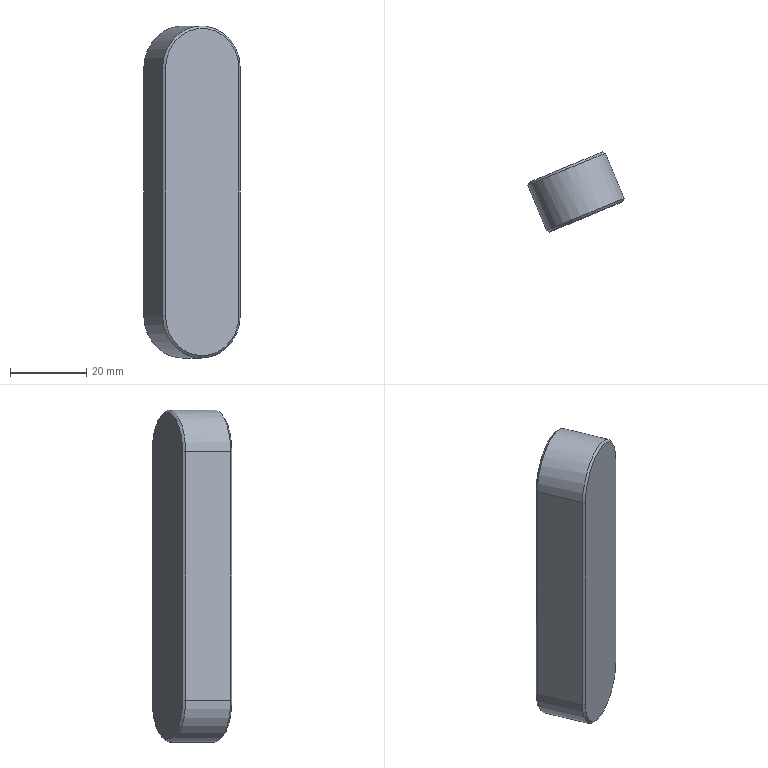Component | SolidWorks | PartAssemblyInLowerHousing-1_LowSpeedAxisAssembly-1_KeyOnLargeGear-1 | 1 solid | 17 faces | box 25.23 x 20.9 x 87 mm | volume 25271 mm3 | plane 8 | cone 6 | cylinder 3 | commonest cylinder face diameters 22 x3 | material Plain Carbon Steel
build123d program:
from build123d import *

# Parameters (mm, degrees)
BOSS_EXTRUDE1_DEPTH = 7
CHAMFER1_SIZE       = 0.6


with BuildPart() as part:
    # Sketch1 → Boss-Extrude1 (new, symmetric)
    with BuildSketch(Plane.XY):
        with BuildLine():
            Line((-26.426, 14.369), (38.574, 14.369))
            ThreePointArc((38.574, 14.369), (49.574, 3.369), (38.574, -7.631))
            Line((38.574, -7.631), (-26.426, -7.631))
            ThreePointArc((-26.426, -7.631), (-37.426, 3.369), (-26.426, 14.369))
        make_face()
    extrude(amount=BOSS_EXTRUDE1_DEPTH, both=True)

    # Chamfer1
    chamfer1_edges = [part.edges().sort_by_distance(p)[0] for p in [
        (49.574, 3.369, 7),
        (6.074, 14.369, 7),
        (-37.426, 3.369, 7),
        (6.074, 14.369, -7),
        (49.574, 3.369, -7),
        (6.074, -7.631, -7),
        (-37.426, 3.369, -7),
        (6.074, -7.631, 7),
    ]]
    chamfer(chamfer1_edges, length=CHAMFER1_SIZE)


solid = part.part

# Placed as in the assembly
solid = solid.moved(Location((1122.204, 1304.711, 1585.639), (-90, -22.523, -90)))
STEP:
#1=COLOUR_RGB('',0.7922,0.8196,0.9333);
#2=FILL_AREA_STYLE_COLOUR('',#1);
#3=FILL_AREA_STYLE('',(#2));
#4=SURFACE_STYLE_FILL_AREA(#3);
#5=SURFACE_SIDE_STYLE('',(#4));
#6=SURFACE_STYLE_USAGE(.BOTH.,#5);
#7=PRESENTATION_STYLE_ASSIGNMENT((#6));
#8=CARTESIAN_POINT('',(44.409,51.163,60.977));
#9=VERTEX_POINT('',#8);
#10=CARTESIAN_POINT('',(44.788,51.32,61.386));
#11=VERTEX_POINT('',#10);
#12=CARTESIAN_POINT('',(44.409,51.163,61.386));
#13=DIRECTION('',(0.383,-0.9237,0.));
#14=DIRECTION('',(0.,0.,-1.));
#15=AXIS2_PLACEMENT_3D('',#12,#13,#14);
#16=CIRCLE('',#15,0.4094);
#17=EDGE_CURVE('',#9,#11,#16,.T.);
#18=ORIENTED_EDGE('',*,*,#17,.F.);
#19=CARTESIAN_POINT('',(44.4,51.185,60.953));
#20=VERTEX_POINT('',#19);
#21=CARTESIAN_POINT('',(44.409,51.163,60.977));
#22=DIRECTION('',(-0.2709,0.6532,-0.7071));
#23=VECTOR('',#22,39.37);
#24=LINE('',#21,#23);
#25=EDGE_CURVE('',#9,#20,#24,.T.);
#26=ORIENTED_EDGE('',*,*,#25,.T.);
#27=CARTESIAN_POINT('',(44.8,51.351,61.386));
#28=VERTEX_POINT('',#27);
#29=CARTESIAN_POINT('',(44.4,51.185,61.386));
#30=DIRECTION('',(-0.383,0.9237,-0.));
#31=DIRECTION('',(0.,0.,-1.));
#32=AXIS2_PLACEMENT_3D('',#29,#30,#31);
#33=CIRCLE('',#32,0.4331);
#34=EDGE_CURVE('',#28,#20,#33,.T.);
#35=ORIENTED_EDGE('',*,*,#34,.F.);
#36=CARTESIAN_POINT('',(44.8,51.351,61.386));
#37=DIRECTION('',(-0.3823,-0.924,0.));
#38=VECTOR('',#37,39.37);
#39=LINE('',#36,#38);
#40=EDGE_CURVE('',#28,#11,#39,.T.);
#41=ORIENTED_EDGE('',*,*,#40,.T.);
#42=EDGE_LOOP('',(#18,#26,#35,#41));
#43=FACE_OUTER_BOUND('',#42,.T.);
#44=CARTESIAN_POINT('',(44.409,51.163,61.386));
#45=DIRECTION('',(-0.383,0.9237,-0.));
#46=DIRECTION('',(0.,0.,-1.));
#47=AXIS2_PLACEMENT_3D('',#44,#45,#46);
#48=CONICAL_SURFACE('',#47,0.4094,0.7854);
#49=ADVANCED_FACE('',(#43),#48,.T.);
#50=CARTESIAN_POINT('',(44.198,51.672,64.355));
#51=VERTEX_POINT('',#50);
#52=CARTESIAN_POINT('',(44.576,51.829,63.945));
#53=VERTEX_POINT('',#52);
#54=CARTESIAN_POINT('',(44.198,51.672,63.945));
#55=DIRECTION('',(-0.383,0.9237,-0.));
#56=DIRECTION('',(0.,0.,-1.));
#57=AXIS2_PLACEMENT_3D('',#54,#55,#56);
#58=CIRCLE('',#57,0.4094);
#59=EDGE_CURVE('',#51,#53,#58,.T.);
#60=ORIENTED_EDGE('',*,*,#59,.F.);
#61=CARTESIAN_POINT('',(44.207,51.65,64.378));
#62=VERTEX_POINT('',#61);
#63=CARTESIAN_POINT('',(44.207,51.65,64.378));
#64=DIRECTION('',(0.2709,-0.6532,0.7071));
#65=VECTOR('',#64,39.37);
#66=LINE('',#63,#65);
#67=EDGE_CURVE('',#51,#62,#66,.T.);
#68=ORIENTED_EDGE('',*,*,#67,.T.);
#69=CARTESIAN_POINT('',(44.607,51.816,63.945));
#70=VERTEX_POINT('',#69);
#71=CARTESIAN_POINT('',(44.207,51.65,63.945));
#72=DIRECTION('',(0.383,-0.9237,0.));
#73=DIRECTION('',(0.,0.,-1.));
#74=AXIS2_PLACEMENT_3D('',#71,#72,#73);
#75=CIRCLE('',#74,0.4331);
#76=EDGE_CURVE('',#70,#62,#75,.T.);
#77=ORIENTED_EDGE('',*,*,#76,.F.);
#78=CARTESIAN_POINT('',(44.576,51.829,63.945));
#79=DIRECTION('',(0.924,-0.3823,0.));
#80=VECTOR('',#79,39.37);
#81=LINE('',#78,#80);
#82=EDGE_CURVE('',#53,#70,#81,.T.);
#83=ORIENTED_EDGE('',*,*,#82,.F.);
#84=EDGE_LOOP('',(#60,#68,#77,#83));
#85=FACE_OUTER_BOUND('',#84,.T.);
#86=CARTESIAN_POINT('',(44.207,51.65,63.945));
#87=DIRECTION('',(0.383,-0.9237,0.));
#88=DIRECTION('',(0.,0.,1.));
#89=AXIS2_PLACEMENT_3D('',#86,#87,#88);
#90=CONICAL_SURFACE('',#89,0.4331,0.7854);
#91=ADVANCED_FACE('',(#85),#90,.T.);
#92=ORIENTED_EDGE('',*,*,#34,.T.);
#93=CARTESIAN_POINT('',(44.207,51.65,60.953));
#94=VERTEX_POINT('',#93);
#95=CARTESIAN_POINT('',(44.409,51.163,60.953));
#96=DIRECTION('',(-0.383,0.9237,-0.));
#97=VECTOR('',#96,39.37);
#98=LINE('',#95,#97);
#99=EDGE_CURVE('',#20,#94,#98,.T.);
#100=ORIENTED_EDGE('',*,*,#99,.T.);
#101=CARTESIAN_POINT('',(44.607,51.816,61.386));
#102=VERTEX_POINT('',#101);
#103=CARTESIAN_POINT('',(44.207,51.65,61.386));
#104=DIRECTION('',(0.383,-0.9237,0.));
#105=DIRECTION('',(0.,0.,-1.));
#106=AXIS2_PLACEMENT_3D('',#103,#104,#105);
#107=CIRCLE('',#106,0.4331);
#108=EDGE_CURVE('',#94,#102,#107,.T.);
#109=ORIENTED_EDGE('',*,*,#108,.T.);
#110=CARTESIAN_POINT('',(44.809,51.329,61.386));
#111=DIRECTION('',(-0.383,0.9237,-0.));
#112=VECTOR('',#111,39.37);
#113=LINE('',#110,#112);
#114=EDGE_CURVE('',#28,#102,#113,.T.);
#115=ORIENTED_EDGE('',*,*,#114,.F.);
#116=EDGE_LOOP('',(#92,#100,#109,#115));
#117=FACE_OUTER_BOUND('',#116,.T.);
#118=CARTESIAN_POINT('',(44.409,51.163,61.386));
#119=DIRECTION('',(-0.383,0.9237,-0.));
#120=DIRECTION('',(0.,0.,-1.));
#121=AXIS2_PLACEMENT_3D('',#118,#119,#120);
#122=CYLINDRICAL_SURFACE('',#121,0.4331);
#123=ADVANCED_FACE('',(#117),#122,.T.);
#124=ORIENTED_EDGE('',*,*,#99,.F.);
#125=CARTESIAN_POINT('',(44.,51.019,61.386));
#126=VERTEX_POINT('',#125);
#127=CARTESIAN_POINT('',(44.4,51.185,61.386));
#128=DIRECTION('',(-0.383,0.9237,-0.));
#129=DIRECTION('',(0.,0.,-1.));
#130=AXIS2_PLACEMENT_3D('',#127,#128,#129);
#131=CIRCLE('',#130,0.4331);
#132=EDGE_CURVE('',#20,#126,#131,.T.);
#133=ORIENTED_EDGE('',*,*,#132,.T.);
#134=CARTESIAN_POINT('',(43.807,51.484,61.386));
#135=VERTEX_POINT('',#134);
#136=CARTESIAN_POINT('',(44.009,50.997,61.386));
#137=DIRECTION('',(-0.383,0.9237,-0.));
#138=VECTOR('',#137,39.37);
#139=LINE('',#136,#138);
#140=EDGE_CURVE('',#126,#135,#139,.T.);
#141=ORIENTED_EDGE('',*,*,#140,.T.);
#142=CARTESIAN_POINT('',(44.207,51.65,61.386));
#143=DIRECTION('',(0.383,-0.9237,0.));
#144=DIRECTION('',(0.,0.,-1.));
#145=AXIS2_PLACEMENT_3D('',#142,#143,#144);
#146=CIRCLE('',#145,0.4331);
#147=EDGE_CURVE('',#135,#94,#146,.T.);
#148=ORIENTED_EDGE('',*,*,#147,.T.);
#149=EDGE_LOOP('',(#124,#133,#141,#148));
#150=FACE_OUTER_BOUND('',#149,.T.);
#151=CARTESIAN_POINT('',(44.409,51.163,61.386));
#152=DIRECTION('',(-0.383,0.9237,-0.));
#153=DIRECTION('',(0.,0.,-1.));
#154=AXIS2_PLACEMENT_3D('',#151,#152,#153);
#155=CYLINDRICAL_SURFACE('',#154,0.4331);
#156=ADVANCED_FACE('',(#150),#155,.T.);
#157=ORIENTED_EDGE('',*,*,#114,.T.);
#158=CARTESIAN_POINT('',(44.607,51.816,63.945));
#159=DIRECTION('',(-0.,0.,1.));
#160=VECTOR('',#159,39.37);
#161=LINE('',#158,#160);
#162=EDGE_CURVE('',#102,#70,#161,.T.);
#163=ORIENTED_EDGE('',*,*,#162,.T.);
#164=CARTESIAN_POINT('',(44.8,51.351,63.945));
#165=VERTEX_POINT('',#164);
#166=CARTESIAN_POINT('',(44.809,51.329,63.945));
#167=DIRECTION('',(-0.383,0.9237,-0.));
#168=VECTOR('',#167,39.37);
#169=LINE('',#166,#168);
#170=EDGE_CURVE('',#165,#70,#169,.T.);
#171=ORIENTED_EDGE('',*,*,#170,.F.);
#172=CARTESIAN_POINT('',(44.8,51.351,63.945));
#173=DIRECTION('',(0.,-0.,-1.));
#174=VECTOR('',#173,39.37);
#175=LINE('',#172,#174);
#176=EDGE_CURVE('',#165,#28,#175,.T.);
#177=ORIENTED_EDGE('',*,*,#176,.T.);
#178=EDGE_LOOP('',(#157,#163,#171,#177));
#179=FACE_OUTER_BOUND('',#178,.T.);
#180=CARTESIAN_POINT('',(44.809,51.329,63.945));
#181=DIRECTION('',(-0.9237,-0.383,-0.));
#182=DIRECTION('',(0.,-0.,-1.));
#183=AXIS2_PLACEMENT_3D('',#180,#181,#182);
#184=PLANE('',#183);
#185=ADVANCED_FACE('',(#179),#184,.F.);
#186=ORIENTED_EDGE('',*,*,#170,.T.);
#187=ORIENTED_EDGE('',*,*,#76,.T.);
#188=CARTESIAN_POINT('',(43.807,51.484,63.945));
#189=VERTEX_POINT('',#188);
#190=CARTESIAN_POINT('',(44.207,51.65,63.945));
#191=DIRECTION('',(0.383,-0.9237,0.));
#192=DIRECTION('',(0.,0.,-1.));
#193=AXIS2_PLACEMENT_3D('',#190,#191,#192);
#194=CIRCLE('',#193,0.4331);
#195=EDGE_CURVE('',#62,#189,#194,.T.);
#196=ORIENTED_EDGE('',*,*,#195,.T.);
#197=CARTESIAN_POINT('',(44.,51.019,63.945));
#198=VERTEX_POINT('',#197);
#199=CARTESIAN_POINT('',(44.009,50.997,63.945));
#200=DIRECTION('',(-0.383,0.9237,-0.));
#201=VECTOR('',#200,39.37);
#202=LINE('',#199,#201);
#203=EDGE_CURVE('',#198,#189,#202,.T.);
#204=ORIENTED_EDGE('',*,*,#203,.F.);
#205=CARTESIAN_POINT('',(44.4,51.185,63.945));
#206=DIRECTION('',(-0.383,0.9237,-0.));
#207=DIRECTION('',(0.,0.,-1.));
#208=AXIS2_PLACEMENT_3D('',#205,#206,#207);
#209=CIRCLE('',#208,0.4331);
#210=EDGE_CURVE('',#198,#165,#209,.T.);
#211=ORIENTED_EDGE('',*,*,#210,.T.);
#212=EDGE_LOOP('',(#186,#187,#196,#204,#211));
#213=FACE_OUTER_BOUND('',#212,.T.);
#214=CARTESIAN_POINT('',(44.409,51.163,63.945));
#215=DIRECTION('',(-0.383,0.9237,-0.));
#216=DIRECTION('',(0.,0.,-1.));
#217=AXIS2_PLACEMENT_3D('',#214,#215,#216);
#218=CYLINDRICAL_SURFACE('',#217,0.4331);
#219=ADVANCED_FACE('',(#213),#218,.T.);
#220=ORIENTED_EDGE('',*,*,#203,.T.);
#221=CARTESIAN_POINT('',(43.807,51.484,61.386));
#222=DIRECTION('',(0.,-0.,-1.));
#223=VECTOR('',#222,39.37);
#224=LINE('',#221,#223);
#225=EDGE_CURVE('',#189,#135,#224,.T.);
#226=ORIENTED_EDGE('',*,*,#225,.T.);
#227=ORIENTED_EDGE('',*,*,#140,.F.);
#228=CARTESIAN_POINT('',(44.,51.019,61.386));
#229=DIRECTION('',(-0.,0.,1.));
#230=VECTOR('',#229,39.37);
#231=LINE('',#228,#230);
#232=EDGE_CURVE('',#126,#198,#231,.T.);
#233=ORIENTED_EDGE('',*,*,#232,.T.);
#234=EDGE_LOOP('',(#220,#226,#227,#233));
#235=FACE_OUTER_BOUND('',#234,.T.);
#236=CARTESIAN_POINT('',(44.009,50.997,61.386));
#237=DIRECTION('',(0.9237,0.383,0.));
#238=DIRECTION('',(-0.,0.,1.));
#239=AXIS2_PLACEMENT_3D('',#236,#237,#238);
#240=PLANE('',#239);
#241=ADVANCED_FACE('',(#235),#240,.F.);
#242=CARTESIAN_POINT('',(44.031,51.006,63.945));
#243=VERTEX_POINT('',#242);
#244=CARTESIAN_POINT('',(44.031,51.006,61.386));
#245=VERTEX_POINT('',#244);
#246=CARTESIAN_POINT('',(44.031,51.006,61.386));
#247=DIRECTION('',(0.,-0.,-1.));
#248=VECTOR('',#247,39.37);
#249=LINE('',#246,#248);
#250=EDGE_CURVE('',#243,#245,#249,.T.);
#251=ORIENTED_EDGE('',*,*,#250,.T.);
#252=CARTESIAN_POINT('',(44.409,51.163,61.386));
#253=DIRECTION('',(0.383,-0.9237,0.));
#254=DIRECTION('',(0.,0.,-1.));
#255=AXIS2_PLACEMENT_3D('',#252,#253,#254);
#256=CIRCLE('',#255,0.4094);
#257=EDGE_CURVE('',#245,#9,#256,.T.);
#258=ORIENTED_EDGE('',*,*,#257,.T.);
#259=ORIENTED_EDGE('',*,*,#17,.T.);
#260=CARTESIAN_POINT('',(44.788,51.32,63.945));
#261=VERTEX_POINT('',#260);
#262=CARTESIAN_POINT('',(44.788,51.32,61.386));
#263=DIRECTION('',(-0.,0.,1.));
#264=VECTOR('',#263,39.37);
#265=LINE('',#262,#264);
#266=EDGE_CURVE('',#11,#261,#265,.T.);
#267=ORIENTED_EDGE('',*,*,#266,.T.);
#268=CARTESIAN_POINT('',(44.409,51.163,63.945));
#269=DIRECTION('',(0.383,-0.9237,0.));
#270=DIRECTION('',(0.,0.,-1.));
#271=AXIS2_PLACEMENT_3D('',#268,#269,#270);
#272=CIRCLE('',#271,0.4094);
#273=EDGE_CURVE('',#261,#243,#272,.T.);
#274=ORIENTED_EDGE('',*,*,#273,.T.);
#275=EDGE_LOOP('',(#251,#258,#259,#267,#274));
#276=FACE_OUTER_BOUND('',#275,.T.);
#277=CARTESIAN_POINT('',(44.409,51.163,61.386));
#278=DIRECTION('',(-0.383,0.9237,-0.));
#279=DIRECTION('',(-0.,-0.,-1.));
#280=AXIS2_PLACEMENT_3D('',#277,#278,#279);
#281=PLANE('',#280);
#282=ADVANCED_FACE('',(#276),#281,.F.);
#283=CARTESIAN_POINT('',(44.576,51.829,61.386));
#284=VERTEX_POINT('',#283);
#285=CARTESIAN_POINT('',(44.576,51.829,61.386));
#286=DIRECTION('',(0.,-0.,-1.));
#287=VECTOR('',#286,39.37);
#288=LINE('',#285,#287);
#289=EDGE_CURVE('',#53,#284,#288,.T.);
#290=ORIENTED_EDGE('',*,*,#289,.T.);
#291=CARTESIAN_POINT('',(43.82,51.515,61.386));
#292=VERTEX_POINT('',#291);
#293=CARTESIAN_POINT('',(44.198,51.672,61.386));
#294=DIRECTION('',(-0.383,0.9237,-0.));
#295=DIRECTION('',(0.,0.,-1.));
#296=AXIS2_PLACEMENT_3D('',#293,#294,#295);
#297=CIRCLE('',#296,0.4094);
#298=EDGE_CURVE('',#284,#292,#297,.T.);
#299=ORIENTED_EDGE('',*,*,#298,.T.);
#300=CARTESIAN_POINT('',(43.82,51.515,63.945));
#301=VERTEX_POINT('',#300);
#302=CARTESIAN_POINT('',(43.82,51.515,63.945));
#303=DIRECTION('',(-0.,0.,1.));
#304=VECTOR('',#303,39.37);
#305=LINE('',#302,#304);
#306=EDGE_CURVE('',#292,#301,#305,.T.);
#307=ORIENTED_EDGE('',*,*,#306,.T.);
#308=CARTESIAN_POINT('',(44.198,51.672,63.945));
#309=DIRECTION('',(-0.383,0.9237,-0.));
#310=DIRECTION('',(0.,0.,-1.));
#311=AXIS2_PLACEMENT_3D('',#308,#309,#310);
#312=CIRCLE('',#311,0.4094);
#313=EDGE_CURVE('',#301,#51,#312,.T.);
#314=ORIENTED_EDGE('',*,*,#313,.T.);
#315=ORIENTED_EDGE('',*,*,#59,.T.);
#316=EDGE_LOOP('',(#290,#299,#307,#314,#315));
#317=FACE_OUTER_BOUND('',#316,.T.);
#318=CARTESIAN_POINT('',(44.198,51.672,61.386));
#319=DIRECTION('',(-0.383,0.9237,-0.));
#320=DIRECTION('',(-0.,-0.,-1.));
#321=AXIS2_PLACEMENT_3D('',#318,#319,#320);
#322=PLANE('',#321);
#323=ADVANCED_FACE('',(#317),#322,.T.);
#324=ORIENTED_EDGE('',*,*,#67,.F.);
#325=ORIENTED_EDGE('',*,*,#313,.F.);
#326=CARTESIAN_POINT('',(43.807,51.484,63.945));
#327=DIRECTION('',(0.3823,0.924,-0.));
#328=VECTOR('',#327,39.37);
#329=LINE('',#326,#328);
#330=EDGE_CURVE('',#189,#301,#329,.T.);
#331=ORIENTED_EDGE('',*,*,#330,.F.);
#332=ORIENTED_EDGE('',*,*,#195,.F.);
#333=EDGE_LOOP('',(#324,#325,#331,#332));
#334=FACE_OUTER_BOUND('',#333,.T.);
#335=CARTESIAN_POINT('',(44.207,51.65,63.945));
#336=DIRECTION('',(0.383,-0.9237,0.));
#337=DIRECTION('',(0.,0.,1.));
#338=AXIS2_PLACEMENT_3D('',#335,#336,#337);
#339=CONICAL_SURFACE('',#338,0.4331,0.7854);
#340=ADVANCED_FACE('',(#334),#339,.T.);
#341=ORIENTED_EDGE('',*,*,#330,.T.);
#342=ORIENTED_EDGE('',*,*,#306,.F.);
#343=CARTESIAN_POINT('',(43.807,51.484,61.386));
#344=DIRECTION('',(0.3823,0.924,-0.));
#345=VECTOR('',#344,39.37);
#346=LINE('',#343,#345);
#347=EDGE_CURVE('',#135,#292,#346,.T.);
#348=ORIENTED_EDGE('',*,*,#347,.F.);
#349=ORIENTED_EDGE('',*,*,#225,.F.);
#350=EDGE_LOOP('',(#341,#342,#348,#349));
#351=FACE_OUTER_BOUND('',#350,.T.);
#352=CARTESIAN_POINT('',(43.807,51.484,61.386));
#353=DIRECTION('',(-0.924,0.3823,-0.));
#354=DIRECTION('',(-0.,0.,1.));
#355=AXIS2_PLACEMENT_3D('',#352,#353,#354);
#356=PLANE('',#355);
#357=ADVANCED_FACE('',(#351),#356,.T.);
#358=ORIENTED_EDGE('',*,*,#82,.T.);
#359=ORIENTED_EDGE('',*,*,#162,.F.);
#360=CARTESIAN_POINT('',(44.576,51.829,61.386));
#361=DIRECTION('',(0.924,-0.3823,0.));
#362=VECTOR('',#361,39.37);
#363=LINE('',#360,#362);
#364=EDGE_CURVE('',#284,#102,#363,.T.);
#365=ORIENTED_EDGE('',*,*,#364,.F.);
#366=ORIENTED_EDGE('',*,*,#289,.F.);
#367=EDGE_LOOP('',(#358,#359,#365,#366));
#368=FACE_OUTER_BOUND('',#367,.T.);
#369=CARTESIAN_POINT('',(44.607,51.816,63.945));
#370=DIRECTION('',(0.3823,0.924,-0.));
#371=DIRECTION('',(0.,-0.,-1.));
#372=AXIS2_PLACEMENT_3D('',#369,#370,#371);
#373=PLANE('',#372);
#374=ADVANCED_FACE('',(#368),#373,.T.);
#375=ORIENTED_EDGE('',*,*,#347,.T.);
#376=ORIENTED_EDGE('',*,*,#298,.F.);
#377=ORIENTED_EDGE('',*,*,#364,.T.);
#378=ORIENTED_EDGE('',*,*,#108,.F.);
#379=ORIENTED_EDGE('',*,*,#147,.F.);
#380=EDGE_LOOP('',(#375,#376,#377,#378,#379));
#381=FACE_OUTER_BOUND('',#380,.T.);
#382=CARTESIAN_POINT('',(44.207,51.65,61.386));
#383=DIRECTION('',(0.383,-0.9237,0.));
#384=DIRECTION('',(0.,0.,1.));
#385=AXIS2_PLACEMENT_3D('',#382,#383,#384);
#386=CONICAL_SURFACE('',#385,0.4331,0.7854);
#387=ADVANCED_FACE('',(#381),#386,.T.);
#388=CARTESIAN_POINT('',(44.8,51.351,63.945));
#389=DIRECTION('',(-0.3823,-0.924,0.));
#390=VECTOR('',#389,39.37);
#391=LINE('',#388,#390);
#392=EDGE_CURVE('',#165,#261,#391,.T.);
#393=ORIENTED_EDGE('',*,*,#392,.F.);
#394=ORIENTED_EDGE('',*,*,#210,.F.);
#395=CARTESIAN_POINT('',(44.031,51.006,63.945));
#396=DIRECTION('',(-0.924,0.3823,-0.));
#397=VECTOR('',#396,39.37);
#398=LINE('',#395,#397);
#399=EDGE_CURVE('',#243,#198,#398,.T.);
#400=ORIENTED_EDGE('',*,*,#399,.F.);
#401=ORIENTED_EDGE('',*,*,#273,.F.);
#402=EDGE_LOOP('',(#393,#394,#400,#401));
#403=FACE_OUTER_BOUND('',#402,.T.);
#404=CARTESIAN_POINT('',(44.409,51.163,63.945));
#405=DIRECTION('',(-0.383,0.9237,-0.));
#406=DIRECTION('',(0.,0.,-1.));
#407=AXIS2_PLACEMENT_3D('',#404,#405,#406);
#408=CONICAL_SURFACE('',#407,0.4094,0.7854);
#409=ADVANCED_FACE('',(#403),#408,.T.);
#410=ORIENTED_EDGE('',*,*,#399,.T.);
#411=ORIENTED_EDGE('',*,*,#232,.F.);
#412=CARTESIAN_POINT('',(44.031,51.006,61.386));
#413=DIRECTION('',(-0.924,0.3823,-0.));
#414=VECTOR('',#413,39.37);
#415=LINE('',#412,#414);
#416=EDGE_CURVE('',#245,#126,#415,.T.);
#417=ORIENTED_EDGE('',*,*,#416,.F.);
#418=ORIENTED_EDGE('',*,*,#250,.F.);
#419=EDGE_LOOP('',(#410,#411,#417,#418));
#420=FACE_OUTER_BOUND('',#419,.T.);
#421=CARTESIAN_POINT('',(44.031,51.006,61.386));
#422=DIRECTION('',(0.3823,0.924,-0.));
#423=DIRECTION('',(0.,-0.,-1.));
#424=AXIS2_PLACEMENT_3D('',#421,#422,#423);
#425=PLANE('',#424);
#426=ADVANCED_FACE('',(#420),#425,.F.);
#427=ORIENTED_EDGE('',*,*,#392,.T.);
#428=ORIENTED_EDGE('',*,*,#266,.F.);
#429=ORIENTED_EDGE('',*,*,#40,.F.);
#430=ORIENTED_EDGE('',*,*,#176,.F.);
#431=EDGE_LOOP('',(#427,#428,#429,#430));
#432=FACE_OUTER_BOUND('',#431,.T.);
#433=CARTESIAN_POINT('',(44.788,51.32,61.386));
#434=DIRECTION('',(-0.924,0.3823,-0.));
#435=DIRECTION('',(-0.,0.,1.));
#436=AXIS2_PLACEMENT_3D('',#433,#434,#435);
#437=PLANE('',#436);
#438=ADVANCED_FACE('',(#432),#437,.F.);
#439=ORIENTED_EDGE('',*,*,#25,.F.);
#440=ORIENTED_EDGE('',*,*,#257,.F.);
#441=ORIENTED_EDGE('',*,*,#416,.T.);
#442=ORIENTED_EDGE('',*,*,#132,.F.);
#443=EDGE_LOOP('',(#439,#440,#441,#442));
#444=FACE_OUTER_BOUND('',#443,.T.);
#445=CARTESIAN_POINT('',(44.409,51.163,61.386));
#446=DIRECTION('',(-0.383,0.9237,-0.));
#447=DIRECTION('',(0.,0.,-1.));
#448=AXIS2_PLACEMENT_3D('',#445,#446,#447);
#449=CONICAL_SURFACE('',#448,0.4094,0.7854);
#450=ADVANCED_FACE('',(#444),#449,.T.);
#451=CLOSED_SHELL('',(#49,#91,#123,#156,#185,#219,#241,#282,#323,#340,#357,#374,#387,#409,#426,#438,#450));
#452=MANIFOLD_SOLID_BREP('',#451);
#453=STYLED_ITEM('',(#7),#452);
#454=(LENGTH_UNIT()NAMED_UNIT(*)SI_UNIT($,.METRE.));
#455=LENGTH_MEASURE_WITH_UNIT(LENGTH_MEASURE(0.0254),#454);
#456=DIMENSIONAL_EXPONENTS(1.,0.,0.,0.,0.,0.,0.);
#457=(CONVERSION_BASED_UNIT('',#455)LENGTH_UNIT()NAMED_UNIT(#456));
#458=UNCERTAINTY_MEASURE_WITH_UNIT(LENGTH_MEASURE(0.00001),#457,'','');
#459=(NAMED_UNIT(*)PLANE_ANGLE_UNIT()SI_UNIT($,.RADIAN.));
#460=(NAMED_UNIT(*)SI_UNIT($,.STERADIAN.)SOLID_ANGLE_UNIT());
#461=(GEOMETRIC_REPRESENTATION_CONTEXT(3)GLOBAL_UNCERTAINTY_ASSIGNED_CONTEXT((#458))GLOBAL_UNIT_ASSIGNED_CONTEXT((#457,#459,#460))REPRESENTATION_CONTEXT('',''));
#462=MECHANICAL_DESIGN_GEOMETRIC_PRESENTATION_REPRESENTATION('',(#453),#461);
#463=CARTESIAN_POINT('',(0.,0.,0.));
#464=DIRECTION('',(0.,0.,1.));
#465=DIRECTION('',(1.,0.,0.));
#466=AXIS2_PLACEMENT_3D('',#463,#464,#465);
#467=(LENGTH_UNIT()NAMED_UNIT(*)SI_UNIT($,.METRE.));
#468=LENGTH_MEASURE_WITH_UNIT(LENGTH_MEASURE(0.0254),#467);
#469=DIMENSIONAL_EXPONENTS(1.,0.,0.,0.,0.,0.,0.);
#470=(CONVERSION_BASED_UNIT('',#468)LENGTH_UNIT()NAMED_UNIT(#469));
#471=UNCERTAINTY_MEASURE_WITH_UNIT(LENGTH_MEASURE(0.00001),#470,'','');
#472=(NAMED_UNIT(*)PLANE_ANGLE_UNIT()SI_UNIT($,.RADIAN.));
#473=(NAMED_UNIT(*)SI_UNIT($,.STERADIAN.)SOLID_ANGLE_UNIT());
#474=(GEOMETRIC_REPRESENTATION_CONTEXT(3)GLOBAL_UNCERTAINTY_ASSIGNED_CONTEXT((#471))GLOBAL_UNIT_ASSIGNED_CONTEXT((#470,#472,#473))REPRESENTATION_CONTEXT('',''));
#475=ADVANCED_BREP_SHAPE_REPRESENTATION('',(#452,#466),#474);
#476=PRESENTATION_LAYER_ASSIGNMENT('','',(#453));